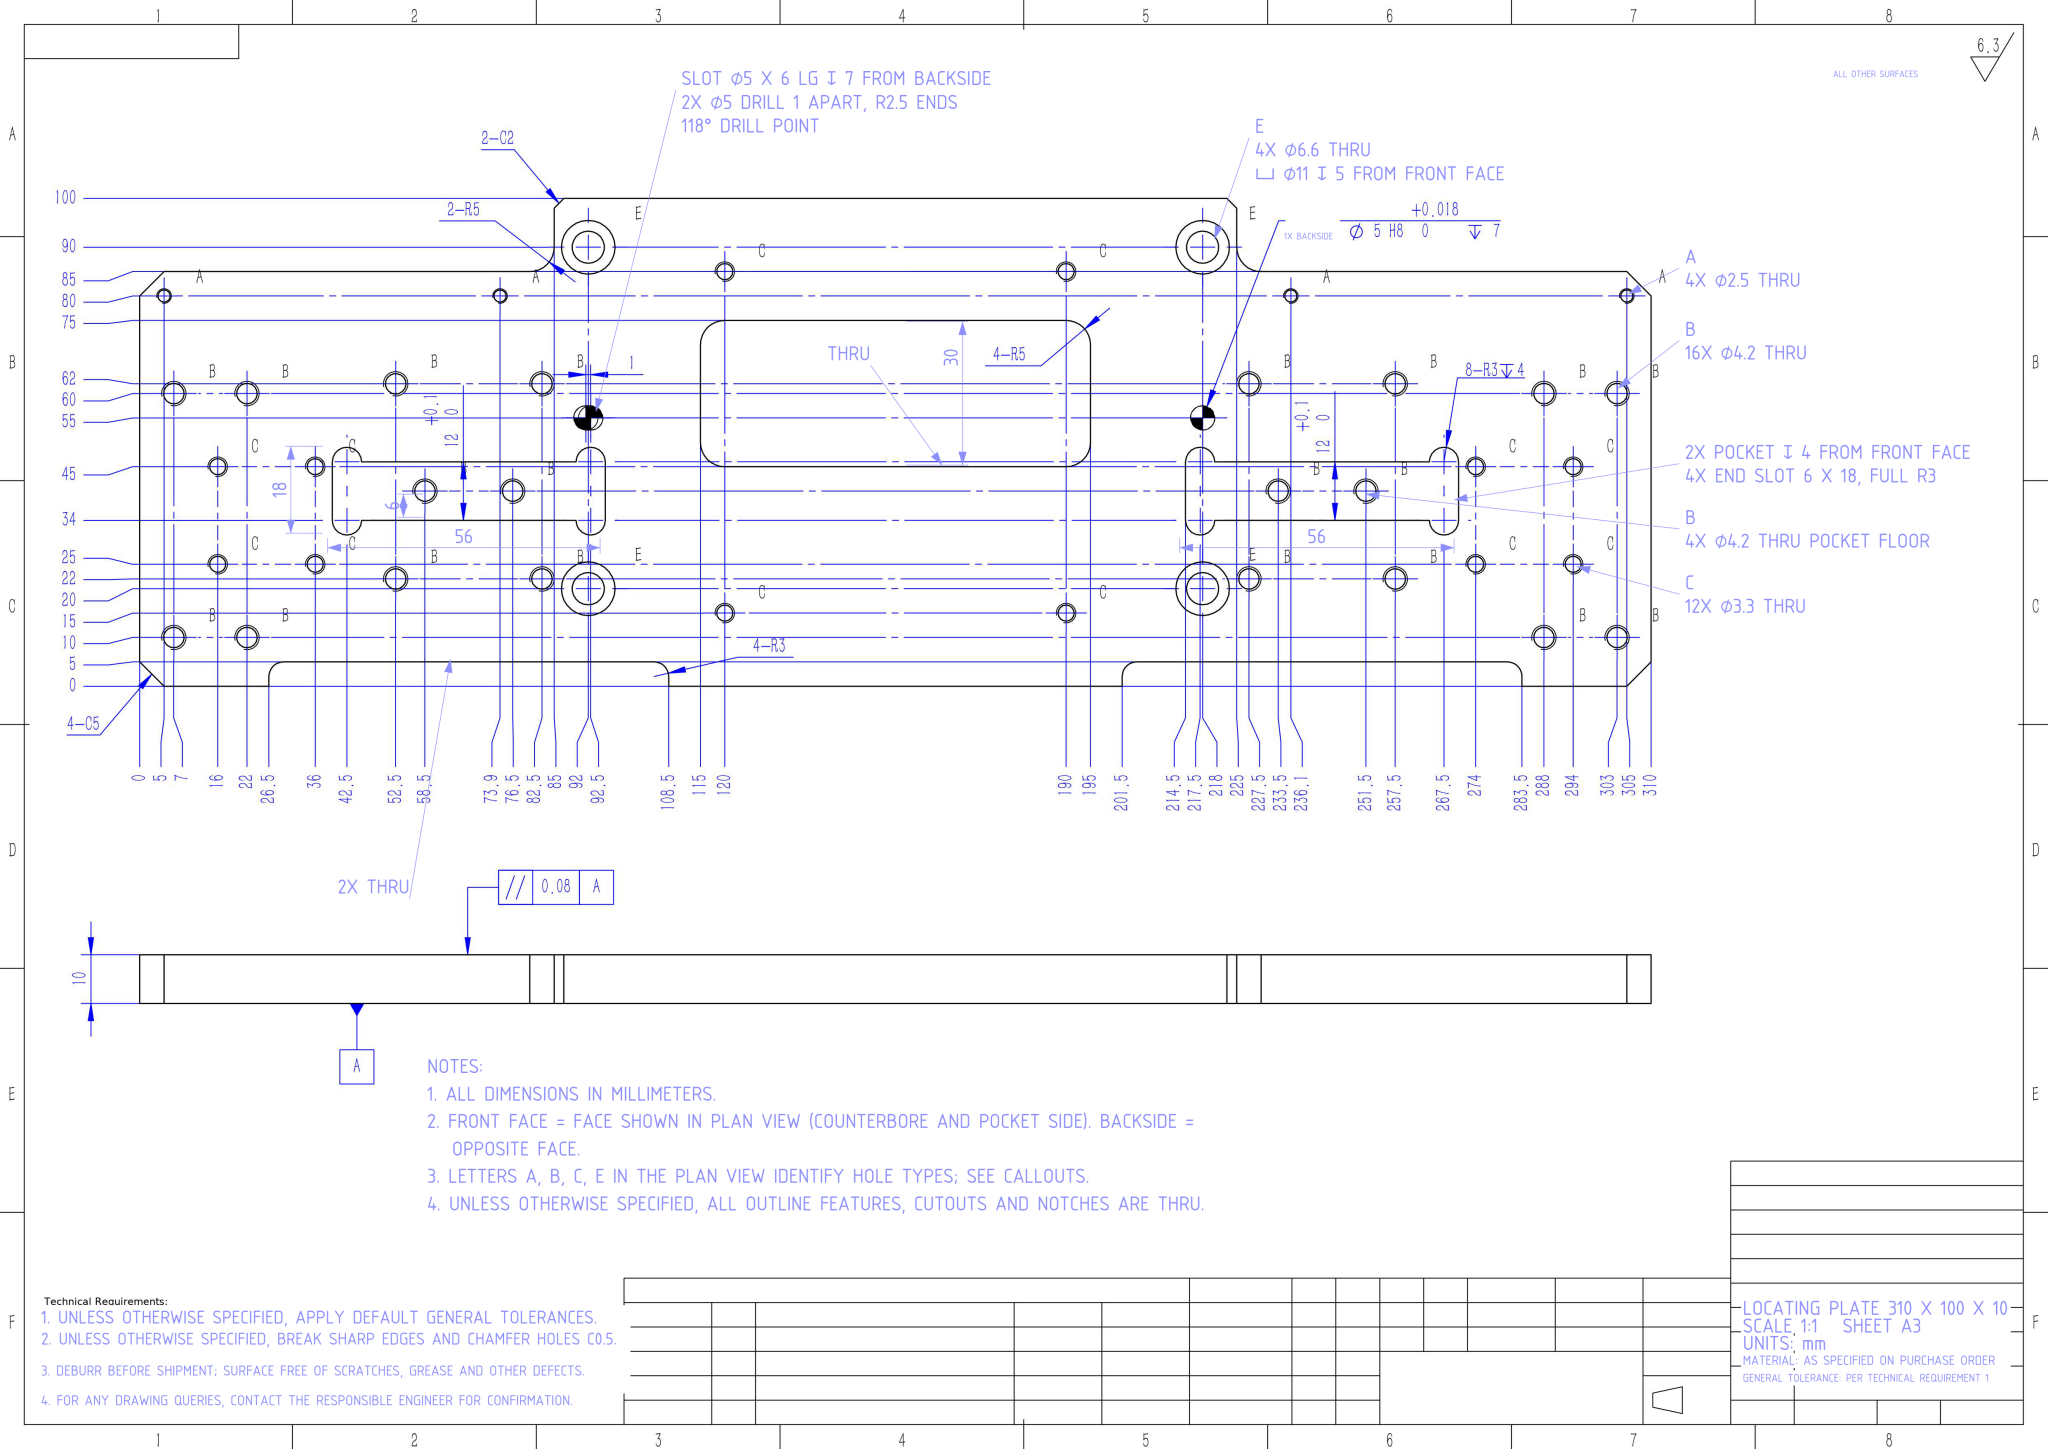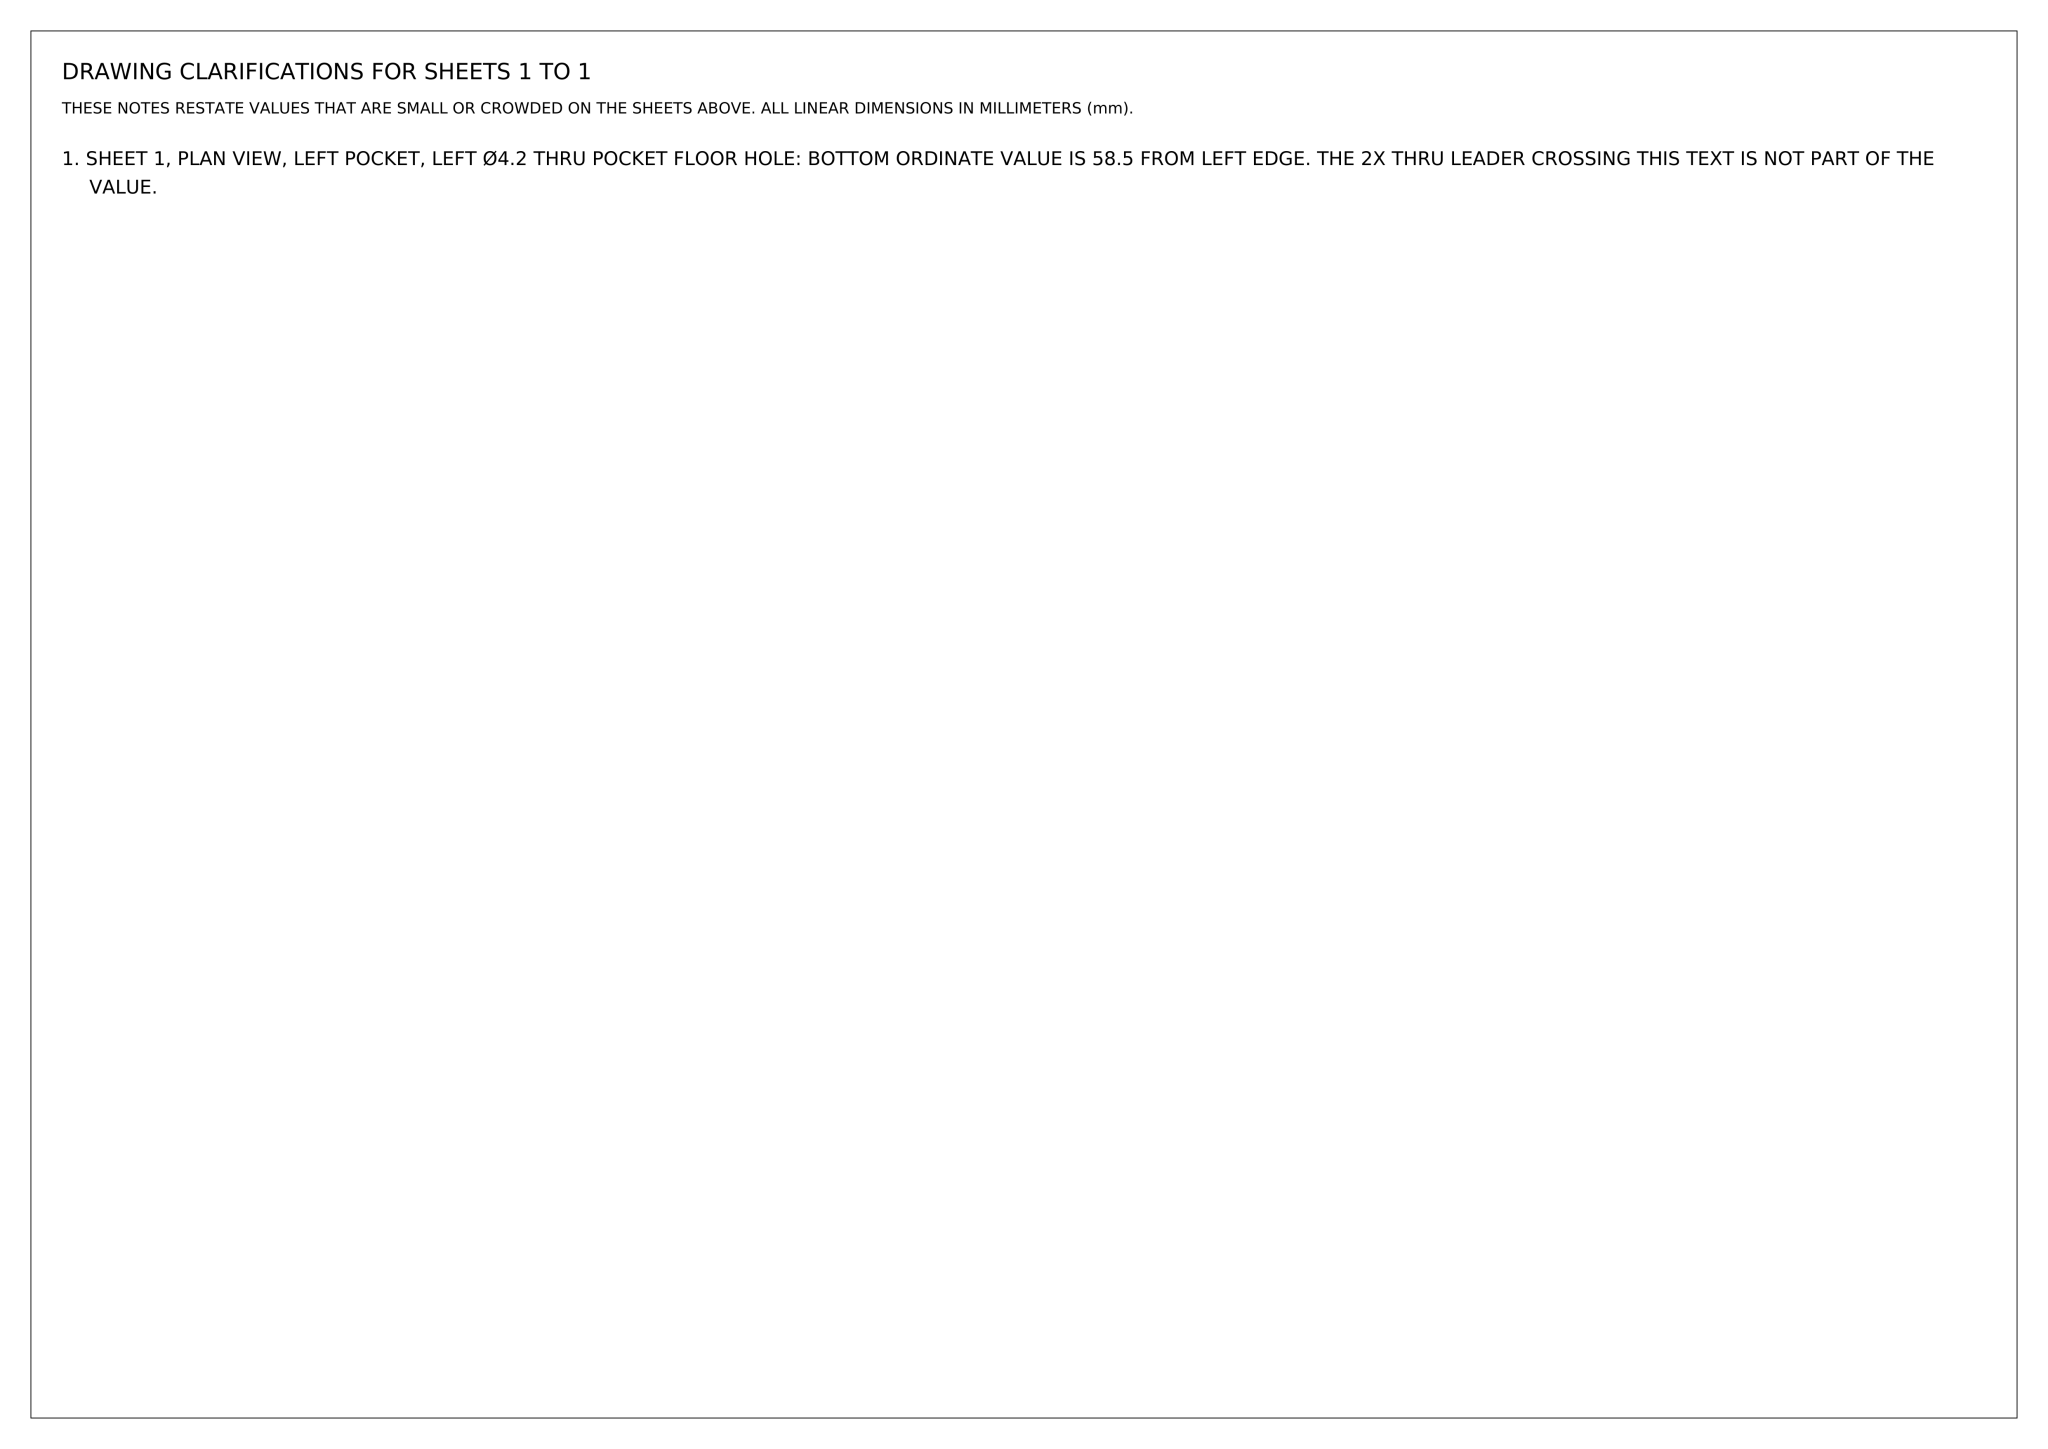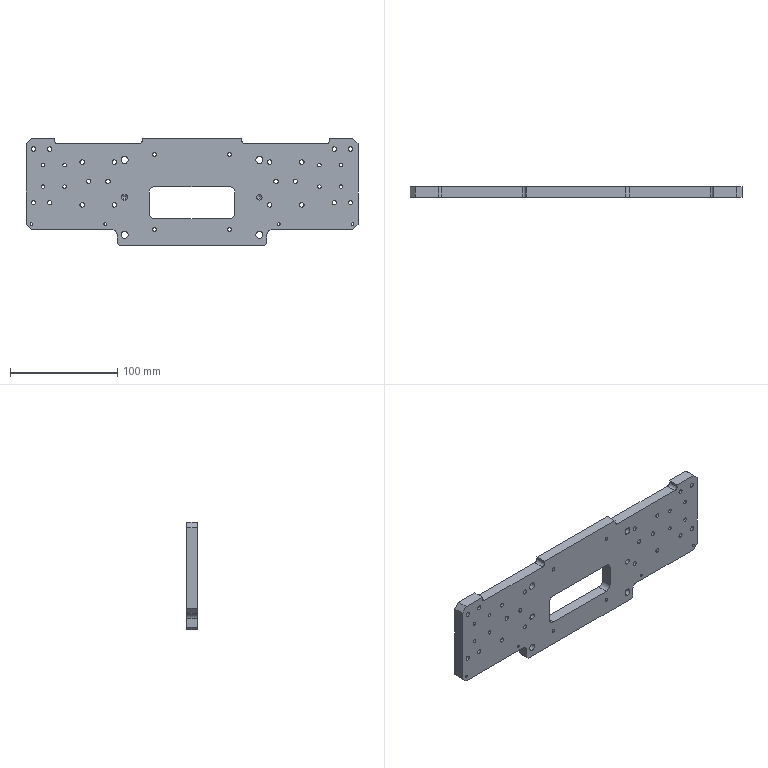Part | NX | mm | 1 solid | 164 faces | box 310 x 10 x 100 mm | volume 239641 mm3 | cylinder 114 | plane 46 | cone 4 | commonest cylinder face diameters 4.2 x40 3.3 x24 6 x16 2.5 x8 11 x8 6.6 x8 10 x6 5 x4